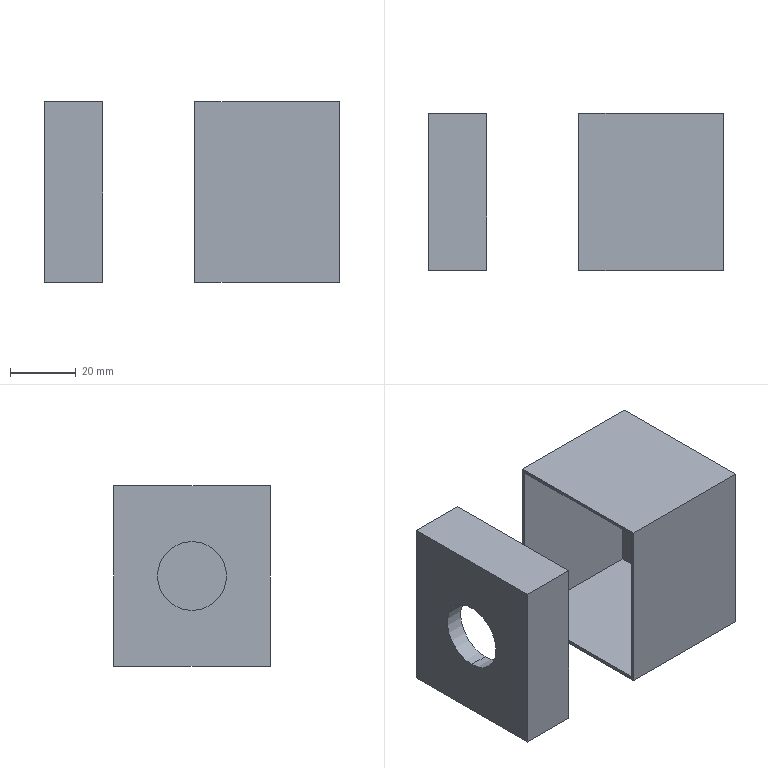Component | SolidWorks | BearingHousing-1 | 2 solids | 24 faces | box 89.77 x 47.79 x 55 mm | volume 29299 mm3 | plane 22 | cylinder 2 | commonest cylinder face diameters 21 x2
STEP:
#1=COLOUR_RGB('',0.7922,0.8196,0.9333);
#2=FILL_AREA_STYLE_COLOUR('',#1);
#3=FILL_AREA_STYLE('',(#2));
#4=SURFACE_STYLE_FILL_AREA(#3);
#5=SURFACE_SIDE_STYLE('',(#4));
#6=SURFACE_STYLE_USAGE(.BOTH.,#5);
#7=PRESENTATION_STYLE_ASSIGNMENT((#6));
#8=CARTESIAN_POINT('',(7.039,3.272,1.043));
#9=VERTEX_POINT('',#8);
#10=CARTESIAN_POINT('',(7.039,1.469,1.043));
#11=VERTEX_POINT('',#10);
#12=CARTESIAN_POINT('',(7.039,3.37,1.043));
#13=DIRECTION('',(0.,-1.,0.));
#14=VECTOR('',#13,39.37);
#15=LINE('',#12,#14);
#16=EDGE_CURVE('',#9,#11,#15,.T.);
#17=ORIENTED_EDGE('',*,*,#16,.T.);
#18=CARTESIAN_POINT('',(7.039,1.469,-1.043));
#19=VERTEX_POINT('',#18);
#20=CARTESIAN_POINT('',(7.039,1.469,0.8331));
#21=DIRECTION('',(-0.,-0.,-1.));
#22=VECTOR('',#21,39.37);
#23=LINE('',#20,#22);
#24=EDGE_CURVE('',#11,#19,#23,.T.);
#25=ORIENTED_EDGE('',*,*,#24,.T.);
#26=CARTESIAN_POINT('',(7.039,3.272,-1.043));
#27=VERTEX_POINT('',#26);
#28=CARTESIAN_POINT('',(7.039,3.37,-1.043));
#29=DIRECTION('',(-0.,1.,-0.));
#30=VECTOR('',#29,39.37);
#31=LINE('',#28,#30);
#32=EDGE_CURVE('',#19,#27,#31,.T.);
#33=ORIENTED_EDGE('',*,*,#32,.T.);
#34=CARTESIAN_POINT('',(7.039,3.272,0.8331));
#35=DIRECTION('',(0.,0.,1.));
#36=VECTOR('',#35,39.37);
#37=LINE('',#34,#36);
#38=EDGE_CURVE('',#27,#9,#37,.T.);
#39=ORIENTED_EDGE('',*,*,#38,.T.);
#40=EDGE_LOOP('',(#17,#25,#33,#39));
#41=FACE_BOUND('',#40,.T.);
#42=CARTESIAN_POINT('',(7.039,1.43,1.083));
#43=VERTEX_POINT('',#42);
#44=CARTESIAN_POINT('',(7.039,1.43,-1.083));
#45=VERTEX_POINT('',#44);
#46=CARTESIAN_POINT('',(7.039,1.43,1.083));
#47=DIRECTION('',(-0.,-0.,-1.));
#48=VECTOR('',#47,39.37);
#49=LINE('',#46,#48);
#50=EDGE_CURVE('',#43,#45,#49,.T.);
#51=ORIENTED_EDGE('',*,*,#50,.F.);
#52=CARTESIAN_POINT('',(7.039,3.312,1.083));
#53=VERTEX_POINT('',#52);
#54=CARTESIAN_POINT('',(7.039,3.312,1.083));
#55=DIRECTION('',(0.,-1.,0.));
#56=VECTOR('',#55,39.37);
#57=LINE('',#54,#56);
#58=EDGE_CURVE('',#53,#43,#57,.T.);
#59=ORIENTED_EDGE('',*,*,#58,.F.);
#60=CARTESIAN_POINT('',(7.039,3.312,-1.083));
#61=VERTEX_POINT('',#60);
#62=CARTESIAN_POINT('',(7.039,3.312,-1.083));
#63=DIRECTION('',(0.,0.,1.));
#64=VECTOR('',#63,39.37);
#65=LINE('',#62,#64);
#66=EDGE_CURVE('',#61,#53,#65,.T.);
#67=ORIENTED_EDGE('',*,*,#66,.F.);
#68=CARTESIAN_POINT('',(7.039,1.43,-1.083));
#69=DIRECTION('',(-0.,1.,-0.));
#70=VECTOR('',#69,39.37);
#71=LINE('',#68,#70);
#72=EDGE_CURVE('',#45,#61,#71,.T.);
#73=ORIENTED_EDGE('',*,*,#72,.F.);
#74=EDGE_LOOP('',(#51,#59,#67,#73));
#75=FACE_OUTER_BOUND('',#74,.T.);
#76=CARTESIAN_POINT('',(7.039,3.37,0.8331));
#77=DIRECTION('',(1.,0.,-0.));
#78=DIRECTION('',(0.,-1.,0.));
#79=AXIS2_PLACEMENT_3D('',#76,#77,#78);
#80=PLANE('',#79);
#81=ADVANCED_FACE('',(#41,#75),#80,.F.);
#82=CARTESIAN_POINT('',(8.771,1.43,-1.083));
#83=VERTEX_POINT('',#82);
#84=CARTESIAN_POINT('',(-2.164,1.43,-1.083));
#85=DIRECTION('',(1.,-0.,0.));
#86=VECTOR('',#85,39.37);
#87=LINE('',#84,#86);
#88=EDGE_CURVE('',#45,#83,#87,.T.);
#89=ORIENTED_EDGE('',*,*,#88,.F.);
#90=ORIENTED_EDGE('',*,*,#72,.T.);
#91=CARTESIAN_POINT('',(8.771,3.312,-1.083));
#92=VERTEX_POINT('',#91);
#93=CARTESIAN_POINT('',(-2.164,3.312,-1.083));
#94=DIRECTION('',(-1.,-0.,-0.));
#95=VECTOR('',#94,39.37);
#96=LINE('',#93,#95);
#97=EDGE_CURVE('',#92,#61,#96,.T.);
#98=ORIENTED_EDGE('',*,*,#97,.F.);
#99=CARTESIAN_POINT('',(8.771,1.43,-1.083));
#100=DIRECTION('',(-0.,1.,-0.));
#101=VECTOR('',#100,39.37);
#102=LINE('',#99,#101);
#103=EDGE_CURVE('',#83,#92,#102,.T.);
#104=ORIENTED_EDGE('',*,*,#103,.F.);
#105=EDGE_LOOP('',(#89,#90,#98,#104));
#106=FACE_OUTER_BOUND('',#105,.T.);
#107=CARTESIAN_POINT('',(-2.164,3.37,-1.083));
#108=DIRECTION('',(-0.,0.,1.));
#109=DIRECTION('',(0.,-1.,0.));
#110=AXIS2_PLACEMENT_3D('',#107,#108,#109);
#111=PLANE('',#110);
#112=ADVANCED_FACE('',(#106),#111,.F.);
#113=ORIENTED_EDGE('',*,*,#58,.T.);
#114=CARTESIAN_POINT('',(8.771,1.43,1.083));
#115=VERTEX_POINT('',#114);
#116=CARTESIAN_POINT('',(-2.164,1.43,1.083));
#117=DIRECTION('',(1.,-0.,0.));
#118=VECTOR('',#117,39.37);
#119=LINE('',#116,#118);
#120=EDGE_CURVE('',#43,#115,#119,.T.);
#121=ORIENTED_EDGE('',*,*,#120,.T.);
#122=CARTESIAN_POINT('',(8.771,3.312,1.083));
#123=VERTEX_POINT('',#122);
#124=CARTESIAN_POINT('',(8.771,3.312,1.083));
#125=DIRECTION('',(0.,-1.,0.));
#126=VECTOR('',#125,39.37);
#127=LINE('',#124,#126);
#128=EDGE_CURVE('',#123,#115,#127,.T.);
#129=ORIENTED_EDGE('',*,*,#128,.F.);
#130=CARTESIAN_POINT('',(-2.164,3.312,1.083));
#131=DIRECTION('',(-1.,-0.,-0.));
#132=VECTOR('',#131,39.37);
#133=LINE('',#130,#132);
#134=EDGE_CURVE('',#123,#53,#133,.T.);
#135=ORIENTED_EDGE('',*,*,#134,.T.);
#136=EDGE_LOOP('',(#113,#121,#129,#135));
#137=FACE_OUTER_BOUND('',#136,.T.);
#138=CARTESIAN_POINT('',(-2.164,3.37,1.083));
#139=DIRECTION('',(-0.,0.,1.));
#140=DIRECTION('',(0.,-1.,0.));
#141=AXIS2_PLACEMENT_3D('',#138,#139,#140);
#142=PLANE('',#141);
#143=ADVANCED_FACE('',(#137),#142,.T.);
#144=ORIENTED_EDGE('',*,*,#120,.F.);
#145=ORIENTED_EDGE('',*,*,#50,.T.);
#146=ORIENTED_EDGE('',*,*,#88,.T.);
#147=CARTESIAN_POINT('',(8.771,1.43,1.083));
#148=DIRECTION('',(-0.,-0.,-1.));
#149=VECTOR('',#148,39.37);
#150=LINE('',#147,#149);
#151=EDGE_CURVE('',#115,#83,#150,.T.);
#152=ORIENTED_EDGE('',*,*,#151,.F.);
#153=EDGE_LOOP('',(#144,#145,#146,#152));
#154=FACE_OUTER_BOUND('',#153,.T.);
#155=CARTESIAN_POINT('',(-2.164,1.43,1.083));
#156=DIRECTION('',(0.,1.,-0.));
#157=DIRECTION('',(0.,0.,1.));
#158=AXIS2_PLACEMENT_3D('',#155,#156,#157);
#159=PLANE('',#158);
#160=ADVANCED_FACE('',(#154),#159,.F.);
#161=ORIENTED_EDGE('',*,*,#97,.T.);
#162=ORIENTED_EDGE('',*,*,#66,.T.);
#163=ORIENTED_EDGE('',*,*,#134,.F.);
#164=CARTESIAN_POINT('',(8.771,3.312,-1.083));
#165=DIRECTION('',(0.,0.,1.));
#166=VECTOR('',#165,39.37);
#167=LINE('',#164,#166);
#168=EDGE_CURVE('',#92,#123,#167,.T.);
#169=ORIENTED_EDGE('',*,*,#168,.F.);
#170=EDGE_LOOP('',(#161,#162,#163,#169));
#171=FACE_OUTER_BOUND('',#170,.T.);
#172=CARTESIAN_POINT('',(-2.164,3.312,1.083));
#173=DIRECTION('',(0.,-1.,0.));
#174=DIRECTION('',(-0.,-0.,-1.));
#175=AXIS2_PLACEMENT_3D('',#172,#173,#174);
#176=PLANE('',#175);
#177=ADVANCED_FACE('',(#171),#176,.F.);
#178=CARTESIAN_POINT('',(8.692,1.469,1.043));
#179=VERTEX_POINT('',#178);
#180=CARTESIAN_POINT('',(8.692,1.469,-1.043));
#181=VERTEX_POINT('',#180);
#182=CARTESIAN_POINT('',(8.692,1.469,1.043));
#183=DIRECTION('',(-0.,-0.,-1.));
#184=VECTOR('',#183,39.37);
#185=LINE('',#182,#184);
#186=EDGE_CURVE('',#179,#181,#185,.T.);
#187=ORIENTED_EDGE('',*,*,#186,.T.);
#188=CARTESIAN_POINT('',(5.464,1.469,-1.043));
#189=DIRECTION('',(1.,0.,0.));
#190=VECTOR('',#189,39.37);
#191=LINE('',#188,#190);
#192=EDGE_CURVE('',#19,#181,#191,.T.);
#193=ORIENTED_EDGE('',*,*,#192,.F.);
#194=ORIENTED_EDGE('',*,*,#24,.F.);
#195=CARTESIAN_POINT('',(5.464,1.469,1.043));
#196=DIRECTION('',(1.,0.,0.));
#197=VECTOR('',#196,39.37);
#198=LINE('',#195,#197);
#199=EDGE_CURVE('',#11,#179,#198,.T.);
#200=ORIENTED_EDGE('',*,*,#199,.T.);
#201=EDGE_LOOP('',(#187,#193,#194,#200));
#202=FACE_OUTER_BOUND('',#201,.T.);
#203=CARTESIAN_POINT('',(5.464,1.469,1.043));
#204=DIRECTION('',(0.,-1.,0.));
#205=DIRECTION('',(-0.,-0.,-1.));
#206=AXIS2_PLACEMENT_3D('',#203,#204,#205);
#207=PLANE('',#206);
#208=ADVANCED_FACE('',(#202),#207,.F.);
#209=CARTESIAN_POINT('',(8.692,3.272,1.043));
#210=VERTEX_POINT('',#209);
#211=CARTESIAN_POINT('',(8.692,3.272,1.043));
#212=DIRECTION('',(0.,-1.,0.));
#213=VECTOR('',#212,39.37);
#214=LINE('',#211,#213);
#215=EDGE_CURVE('',#210,#179,#214,.T.);
#216=ORIENTED_EDGE('',*,*,#215,.T.);
#217=ORIENTED_EDGE('',*,*,#199,.F.);
#218=ORIENTED_EDGE('',*,*,#16,.F.);
#219=CARTESIAN_POINT('',(5.464,3.272,1.043));
#220=DIRECTION('',(1.,0.,0.));
#221=VECTOR('',#220,39.37);
#222=LINE('',#219,#221);
#223=EDGE_CURVE('',#9,#210,#222,.T.);
#224=ORIENTED_EDGE('',*,*,#223,.T.);
#225=EDGE_LOOP('',(#216,#217,#218,#224));
#226=FACE_OUTER_BOUND('',#225,.T.);
#227=CARTESIAN_POINT('',(5.464,3.272,1.043));
#228=DIRECTION('',(-0.,0.,1.));
#229=DIRECTION('',(0.,-1.,0.));
#230=AXIS2_PLACEMENT_3D('',#227,#228,#229);
#231=PLANE('',#230);
#232=ADVANCED_FACE('',(#226),#231,.F.);
#233=CARTESIAN_POINT('',(8.692,3.272,-1.043));
#234=VERTEX_POINT('',#233);
#235=CARTESIAN_POINT('',(8.692,3.272,-1.043));
#236=DIRECTION('',(0.,0.,1.));
#237=VECTOR('',#236,39.37);
#238=LINE('',#235,#237);
#239=EDGE_CURVE('',#234,#210,#238,.T.);
#240=ORIENTED_EDGE('',*,*,#239,.T.);
#241=ORIENTED_EDGE('',*,*,#223,.F.);
#242=ORIENTED_EDGE('',*,*,#38,.F.);
#243=CARTESIAN_POINT('',(5.464,3.272,-1.043));
#244=DIRECTION('',(1.,0.,0.));
#245=VECTOR('',#244,39.37);
#246=LINE('',#243,#245);
#247=EDGE_CURVE('',#27,#234,#246,.T.);
#248=ORIENTED_EDGE('',*,*,#247,.T.);
#249=EDGE_LOOP('',(#240,#241,#242,#248));
#250=FACE_OUTER_BOUND('',#249,.T.);
#251=CARTESIAN_POINT('',(5.464,3.272,-1.043));
#252=DIRECTION('',(-0.,1.,-0.));
#253=DIRECTION('',(0.,0.,1.));
#254=AXIS2_PLACEMENT_3D('',#251,#252,#253);
#255=PLANE('',#254);
#256=ADVANCED_FACE('',(#250),#255,.F.);
#257=CARTESIAN_POINT('',(8.692,1.469,-1.043));
#258=DIRECTION('',(-0.,1.,-0.));
#259=VECTOR('',#258,39.37);
#260=LINE('',#257,#259);
#261=EDGE_CURVE('',#181,#234,#260,.T.);
#262=ORIENTED_EDGE('',*,*,#261,.T.);
#263=ORIENTED_EDGE('',*,*,#247,.F.);
#264=ORIENTED_EDGE('',*,*,#32,.F.);
#265=ORIENTED_EDGE('',*,*,#192,.T.);
#266=EDGE_LOOP('',(#262,#263,#264,#265));
#267=FACE_OUTER_BOUND('',#266,.T.);
#268=CARTESIAN_POINT('',(5.464,1.469,-1.043));
#269=DIRECTION('',(0.,-0.,-1.));
#270=DIRECTION('',(-0.,1.,-0.));
#271=AXIS2_PLACEMENT_3D('',#268,#269,#270);
#272=PLANE('',#271);
#273=ADVANCED_FACE('',(#267),#272,.F.);
#274=ORIENTED_EDGE('',*,*,#151,.T.);
#275=ORIENTED_EDGE('',*,*,#103,.T.);
#276=ORIENTED_EDGE('',*,*,#168,.T.);
#277=ORIENTED_EDGE('',*,*,#128,.T.);
#278=EDGE_LOOP('',(#274,#275,#276,#277));
#279=FACE_OUTER_BOUND('',#278,.T.);
#280=CARTESIAN_POINT('',(8.771,3.37,0.8331));
#281=DIRECTION('',(1.,0.,-0.));
#282=DIRECTION('',(0.,-1.,0.));
#283=AXIS2_PLACEMENT_3D('',#280,#281,#282);
#284=PLANE('',#283);
#285=ADVANCED_FACE('',(#279),#284,.T.);
#286=ORIENTED_EDGE('',*,*,#215,.F.);
#287=ORIENTED_EDGE('',*,*,#239,.F.);
#288=ORIENTED_EDGE('',*,*,#261,.F.);
#289=ORIENTED_EDGE('',*,*,#186,.F.);
#290=EDGE_LOOP('',(#286,#287,#288,#289));
#291=FACE_OUTER_BOUND('',#290,.T.);
#292=CARTESIAN_POINT('',(8.692,3.37,0.8331));
#293=DIRECTION('',(1.,0.,-0.));
#294=DIRECTION('',(0.,-1.,0.));
#295=AXIS2_PLACEMENT_3D('',#292,#293,#294);
#296=PLANE('',#295);
#297=ADVANCED_FACE('',(#291),#296,.F.);
#298=CLOSED_SHELL('',(#81,#112,#143,#160,#177,#208,#232,#256,#273,#285,#297));
#299=MANIFOLD_SOLID_BREP('',#298);
#300=STYLED_ITEM('',(#7),#299);
#301=(LENGTH_UNIT()NAMED_UNIT(*)SI_UNIT($,.METRE.));
#302=LENGTH_MEASURE_WITH_UNIT(LENGTH_MEASURE(0.0254),#301);
#303=DIMENSIONAL_EXPONENTS(1.,0.,0.,0.,0.,0.,0.);
#304=(CONVERSION_BASED_UNIT('',#302)LENGTH_UNIT()NAMED_UNIT(#303));
#305=UNCERTAINTY_MEASURE_WITH_UNIT(LENGTH_MEASURE(0.00001),#304,'','');
#306=(NAMED_UNIT(*)PLANE_ANGLE_UNIT()SI_UNIT($,.RADIAN.));
#307=(NAMED_UNIT(*)SI_UNIT($,.STERADIAN.)SOLID_ANGLE_UNIT());
#308=(GEOMETRIC_REPRESENTATION_CONTEXT(3)GLOBAL_UNCERTAINTY_ASSIGNED_CONTEXT((#305))GLOBAL_UNIT_ASSIGNED_CONTEXT((#304,#306,#307))REPRESENTATION_CONTEXT('',''));
#309=MECHANICAL_DESIGN_GEOMETRIC_PRESENTATION_REPRESENTATION('',(#300),#308);
#310=COLOUR_RGB('',0.7922,0.8196,0.9333);
#311=FILL_AREA_STYLE_COLOUR('',#310);
#312=FILL_AREA_STYLE('',(#311));
#313=SURFACE_STYLE_FILL_AREA(#312);
#314=SURFACE_SIDE_STYLE('',(#313));
#315=SURFACE_STYLE_USAGE(.BOTH.,#314);
#316=PRESENTATION_STYLE_ASSIGNMENT((#315));
#317=CARTESIAN_POINT('',(5.464,2.371,-0.4134));
#318=VERTEX_POINT('',#317);
#319=CARTESIAN_POINT('',(5.464,2.371,0.4134));
#320=VERTEX_POINT('',#319);
#321=CARTESIAN_POINT('',(5.464,2.371,-0.));
#322=DIRECTION('',(-1.,-0.,0.));
#323=DIRECTION('',(0.,-1.,0.));
#324=AXIS2_PLACEMENT_3D('',#321,#322,#323);
#325=CIRCLE('',#324,0.4134);
#326=EDGE_CURVE('',#318,#320,#325,.T.);
#327=ORIENTED_EDGE('',*,*,#326,.F.);
#328=CARTESIAN_POINT('',(5.237,2.371,-0.4134));
#329=VERTEX_POINT('',#328);
#330=CARTESIAN_POINT('',(7.639,2.371,-0.4134));
#331=DIRECTION('',(-1.,-0.,-0.));
#332=VECTOR('',#331,39.37);
#333=LINE('',#330,#332);
#334=EDGE_CURVE('',#318,#329,#333,.T.);
#335=ORIENTED_EDGE('',*,*,#334,.T.);
#336=CARTESIAN_POINT('',(5.237,2.371,0.4134));
#337=VERTEX_POINT('',#336);
#338=CARTESIAN_POINT('',(5.237,2.371,-0.));
#339=DIRECTION('',(-1.,-0.,-0.));
#340=DIRECTION('',(0.,0.,1.));
#341=AXIS2_PLACEMENT_3D('',#338,#339,#340);
#342=CIRCLE('',#341,0.4134);
#343=EDGE_CURVE('',#329,#337,#342,.T.);
#344=ORIENTED_EDGE('',*,*,#343,.T.);
#345=CARTESIAN_POINT('',(7.639,2.371,0.4134));
#346=DIRECTION('',(-1.,-0.,-0.));
#347=VECTOR('',#346,39.37);
#348=LINE('',#345,#347);
#349=EDGE_CURVE('',#320,#337,#348,.T.);
#350=ORIENTED_EDGE('',*,*,#349,.F.);
#351=EDGE_LOOP('',(#327,#335,#344,#350));
#352=FACE_OUTER_BOUND('',#351,.T.);
#353=CARTESIAN_POINT('',(7.639,2.371,0.));
#354=DIRECTION('',(-1.,-0.,-0.));
#355=DIRECTION('',(0.,0.,1.));
#356=AXIS2_PLACEMENT_3D('',#353,#354,#355);
#357=CYLINDRICAL_SURFACE('',#356,0.4134);
#358=ADVANCED_FACE('',(#352),#357,.F.);
#359=CARTESIAN_POINT('',(5.237,1.43,1.083));
#360=VERTEX_POINT('',#359);
#361=CARTESIAN_POINT('',(5.936,1.43,1.083));
#362=VERTEX_POINT('',#361);
#363=CARTESIAN_POINT('',(-2.164,1.43,1.083));
#364=DIRECTION('',(1.,-0.,0.));
#365=VECTOR('',#364,39.37);
#366=LINE('',#363,#365);
#367=EDGE_CURVE('',#360,#362,#366,.T.);
#368=ORIENTED_EDGE('',*,*,#367,.T.);
#369=CARTESIAN_POINT('',(5.936,3.312,1.083));
#370=VERTEX_POINT('',#369);
#371=CARTESIAN_POINT('',(5.936,3.312,1.083));
#372=DIRECTION('',(0.,-1.,0.));
#373=VECTOR('',#372,39.37);
#374=LINE('',#371,#373);
#375=EDGE_CURVE('',#370,#362,#374,.T.);
#376=ORIENTED_EDGE('',*,*,#375,.F.);
#377=CARTESIAN_POINT('',(5.237,3.312,1.083));
#378=VERTEX_POINT('',#377);
#379=CARTESIAN_POINT('',(-2.164,3.312,1.083));
#380=DIRECTION('',(-1.,-0.,-0.));
#381=VECTOR('',#380,39.37);
#382=LINE('',#379,#381);
#383=EDGE_CURVE('',#370,#378,#382,.T.);
#384=ORIENTED_EDGE('',*,*,#383,.T.);
#385=CARTESIAN_POINT('',(5.237,3.37,1.083));
#386=DIRECTION('',(0.,-1.,0.));
#387=VECTOR('',#386,39.37);
#388=LINE('',#385,#387);
#389=EDGE_CURVE('',#378,#360,#388,.T.);
#390=ORIENTED_EDGE('',*,*,#389,.T.);
#391=EDGE_LOOP('',(#368,#376,#384,#390));
#392=FACE_OUTER_BOUND('',#391,.T.);
#393=CARTESIAN_POINT('',(-2.164,3.37,1.083));
#394=DIRECTION('',(-0.,0.,1.));
#395=DIRECTION('',(0.,-1.,0.));
#396=AXIS2_PLACEMENT_3D('',#393,#394,#395);
#397=PLANE('',#396);
#398=ADVANCED_FACE('',(#392),#397,.T.);
#399=CARTESIAN_POINT('',(5.936,3.312,-1.083));
#400=VERTEX_POINT('',#399);
#401=CARTESIAN_POINT('',(5.936,3.312,-1.083));
#402=DIRECTION('',(0.,0.,1.));
#403=VECTOR('',#402,39.37);
#404=LINE('',#401,#403);
#405=EDGE_CURVE('',#400,#370,#404,.T.);
#406=ORIENTED_EDGE('',*,*,#405,.F.);
#407=CARTESIAN_POINT('',(5.237,3.312,-1.083));
#408=VERTEX_POINT('',#407);
#409=CARTESIAN_POINT('',(-2.164,3.312,-1.083));
#410=DIRECTION('',(-1.,-0.,-0.));
#411=VECTOR('',#410,39.37);
#412=LINE('',#409,#411);
#413=EDGE_CURVE('',#400,#408,#412,.T.);
#414=ORIENTED_EDGE('',*,*,#413,.T.);
#415=CARTESIAN_POINT('',(5.237,3.312,1.083));
#416=DIRECTION('',(0.,-0.,-1.));
#417=VECTOR('',#416,39.37);
#418=LINE('',#415,#417);
#419=EDGE_CURVE('',#378,#408,#418,.T.);
#420=ORIENTED_EDGE('',*,*,#419,.F.);
#421=ORIENTED_EDGE('',*,*,#383,.F.);
#422=EDGE_LOOP('',(#406,#414,#420,#421));
#423=FACE_OUTER_BOUND('',#422,.T.);
#424=CARTESIAN_POINT('',(-2.164,3.312,1.083));
#425=DIRECTION('',(0.,-1.,0.));
#426=DIRECTION('',(-0.,-0.,-1.));
#427=AXIS2_PLACEMENT_3D('',#424,#425,#426);
#428=PLANE('',#427);
#429=ADVANCED_FACE('',(#423),#428,.F.);
#430=CARTESIAN_POINT('',(5.936,1.43,-1.083));
#431=VERTEX_POINT('',#430);
#432=CARTESIAN_POINT('',(5.936,1.43,-1.083));
#433=DIRECTION('',(-0.,1.,-0.));
#434=VECTOR('',#433,39.37);
#435=LINE('',#432,#434);
#436=EDGE_CURVE('',#431,#400,#435,.T.);
#437=ORIENTED_EDGE('',*,*,#436,.F.);
#438=CARTESIAN_POINT('',(5.237,1.43,-1.083));
#439=VERTEX_POINT('',#438);
#440=CARTESIAN_POINT('',(-2.164,1.43,-1.083));
#441=DIRECTION('',(1.,-0.,0.));
#442=VECTOR('',#441,39.37);
#443=LINE('',#440,#442);
#444=EDGE_CURVE('',#439,#431,#443,.T.);
#445=ORIENTED_EDGE('',*,*,#444,.F.);
#446=CARTESIAN_POINT('',(5.237,3.37,-1.083));
#447=DIRECTION('',(0.,-1.,0.));
#448=VECTOR('',#447,39.37);
#449=LINE('',#446,#448);
#450=EDGE_CURVE('',#408,#439,#449,.T.);
#451=ORIENTED_EDGE('',*,*,#450,.F.);
#452=ORIENTED_EDGE('',*,*,#413,.F.);
#453=EDGE_LOOP('',(#437,#445,#451,#452));
#454=FACE_OUTER_BOUND('',#453,.T.);
#455=CARTESIAN_POINT('',(-2.164,3.37,-1.083));
#456=DIRECTION('',(-0.,0.,1.));
#457=DIRECTION('',(0.,-1.,0.));
#458=AXIS2_PLACEMENT_3D('',#455,#456,#457);
#459=PLANE('',#458);
#460=ADVANCED_FACE('',(#454),#459,.F.);
#461=CARTESIAN_POINT('',(5.237,2.371,-0.));
#462=DIRECTION('',(-1.,-0.,-0.));
#463=DIRECTION('',(0.,0.,1.));
#464=AXIS2_PLACEMENT_3D('',#461,#462,#463);
#465=CIRCLE('',#464,0.4134);
#466=EDGE_CURVE('',#337,#329,#465,.T.);
#467=ORIENTED_EDGE('',*,*,#466,.F.);
#468=ORIENTED_EDGE('',*,*,#343,.F.);
#469=EDGE_LOOP('',(#467,#468));
#470=FACE_BOUND('',#469,.T.);
#471=ORIENTED_EDGE('',*,*,#450,.T.);
#472=CARTESIAN_POINT('',(5.237,1.43,1.083));
#473=DIRECTION('',(0.,-0.,-1.));
#474=VECTOR('',#473,39.37);
#475=LINE('',#472,#474);
#476=EDGE_CURVE('',#360,#439,#475,.T.);
#477=ORIENTED_EDGE('',*,*,#476,.F.);
#478=ORIENTED_EDGE('',*,*,#389,.F.);
#479=ORIENTED_EDGE('',*,*,#419,.T.);
#480=EDGE_LOOP('',(#471,#477,#478,#479));
#481=FACE_OUTER_BOUND('',#480,.T.);
#482=CARTESIAN_POINT('',(5.237,3.37,1.083));
#483=DIRECTION('',(1.,0.,0.));
#484=DIRECTION('',(0.,-0.,-1.));
#485=AXIS2_PLACEMENT_3D('',#482,#483,#484);
#486=PLANE('',#485);
#487=ADVANCED_FACE('',(#470,#481),#486,.F.);
#488=ORIENTED_EDGE('',*,*,#334,.F.);
#489=CARTESIAN_POINT('',(5.464,2.371,-0.));
#490=DIRECTION('',(-1.,-0.,0.));
#491=DIRECTION('',(0.,-1.,0.));
#492=AXIS2_PLACEMENT_3D('',#489,#490,#491);
#493=CIRCLE('',#492,0.4134);
#494=EDGE_CURVE('',#320,#318,#493,.T.);
#495=ORIENTED_EDGE('',*,*,#494,.F.);
#496=ORIENTED_EDGE('',*,*,#349,.T.);
#497=ORIENTED_EDGE('',*,*,#466,.T.);
#498=EDGE_LOOP('',(#488,#495,#496,#497));
#499=FACE_OUTER_BOUND('',#498,.T.);
#500=CARTESIAN_POINT('',(7.639,2.371,0.));
#501=DIRECTION('',(-1.,-0.,-0.));
#502=DIRECTION('',(0.,0.,1.));
#503=AXIS2_PLACEMENT_3D('',#500,#501,#502);
#504=CYLINDRICAL_SURFACE('',#503,0.4134);
#505=ADVANCED_FACE('',(#499),#504,.F.);
#506=CARTESIAN_POINT('',(5.936,1.43,1.083));
#507=DIRECTION('',(-0.,-0.,-1.));
#508=VECTOR('',#507,39.37);
#509=LINE('',#506,#508);
#510=EDGE_CURVE('',#362,#431,#509,.T.);
#511=ORIENTED_EDGE('',*,*,#510,.F.);
#512=ORIENTED_EDGE('',*,*,#367,.F.);
#513=ORIENTED_EDGE('',*,*,#476,.T.);
#514=ORIENTED_EDGE('',*,*,#444,.T.);
#515=EDGE_LOOP('',(#511,#512,#513,#514));
#516=FACE_OUTER_BOUND('',#515,.T.);
#517=CARTESIAN_POINT('',(-2.164,1.43,1.083));
#518=DIRECTION('',(0.,1.,-0.));
#519=DIRECTION('',(0.,0.,1.));
#520=AXIS2_PLACEMENT_3D('',#517,#518,#519);
#521=PLANE('',#520);
#522=ADVANCED_FACE('',(#516),#521,.F.);
#523=CARTESIAN_POINT('',(5.936,1.469,1.043));
#524=VERTEX_POINT('',#523);
#525=CARTESIAN_POINT('',(5.936,1.469,-1.043));
#526=VERTEX_POINT('',#525);
#527=CARTESIAN_POINT('',(5.936,1.469,0.8331));
#528=DIRECTION('',(-0.,-0.,-1.));
#529=VECTOR('',#528,39.37);
#530=LINE('',#527,#529);
#531=EDGE_CURVE('',#524,#526,#530,.T.);
#532=ORIENTED_EDGE('',*,*,#531,.F.);
#533=CARTESIAN_POINT('',(5.936,3.272,1.043));
#534=VERTEX_POINT('',#533);
#535=CARTESIAN_POINT('',(5.936,3.37,1.043));
#536=DIRECTION('',(0.,-1.,0.));
#537=VECTOR('',#536,39.37);
#538=LINE('',#535,#537);
#539=EDGE_CURVE('',#534,#524,#538,.T.);
#540=ORIENTED_EDGE('',*,*,#539,.F.);
#541=CARTESIAN_POINT('',(5.936,3.272,-1.043));
#542=VERTEX_POINT('',#541);
#543=CARTESIAN_POINT('',(5.936,3.272,0.8331));
#544=DIRECTION('',(0.,0.,1.));
#545=VECTOR('',#544,39.37);
#546=LINE('',#543,#545);
#547=EDGE_CURVE('',#542,#534,#546,.T.);
#548=ORIENTED_EDGE('',*,*,#547,.F.);
#549=CARTESIAN_POINT('',(5.936,3.37,-1.043));
#550=DIRECTION('',(-0.,1.,-0.));
#551=VECTOR('',#550,39.37);
#552=LINE('',#549,#551);
#553=EDGE_CURVE('',#526,#542,#552,.T.);
#554=ORIENTED_EDGE('',*,*,#553,.F.);
#555=EDGE_LOOP('',(#532,#540,#548,#554));
#556=FACE_BOUND('',#555,.T.);
#557=ORIENTED_EDGE('',*,*,#510,.T.);
#558=ORIENTED_EDGE('',*,*,#436,.T.);
#559=ORIENTED_EDGE('',*,*,#405,.T.);
#560=ORIENTED_EDGE('',*,*,#375,.T.);
#561=EDGE_LOOP('',(#557,#558,#559,#560));
#562=FACE_OUTER_BOUND('',#561,.T.);
#563=CARTESIAN_POINT('',(5.936,3.37,0.8331));
#564=DIRECTION('',(1.,0.,-0.));
#565=DIRECTION('',(0.,-1.,0.));
#566=AXIS2_PLACEMENT_3D('',#563,#564,#565);
#567=PLANE('',#566);
#568=ADVANCED_FACE('',(#556,#562),#567,.T.);
#569=CARTESIAN_POINT('',(5.464,1.469,1.043));
#570=VERTEX_POINT('',#569);
#571=CARTESIAN_POINT('',(5.464,1.469,-1.043));
#572=VERTEX_POINT('',#571);
#573=CARTESIAN_POINT('',(5.464,1.469,1.043));
#574=DIRECTION('',(-0.,-0.,-1.));
#575=VECTOR('',#574,39.37);
#576=LINE('',#573,#575);
#577=EDGE_CURVE('',#570,#572,#576,.T.);
#578=ORIENTED_EDGE('',*,*,#577,.T.);
#579=CARTESIAN_POINT('',(5.464,3.272,-1.043));
#580=VERTEX_POINT('',#579);
#581=CARTESIAN_POINT('',(5.464,1.469,-1.043));
#582=DIRECTION('',(-0.,1.,-0.));
#583=VECTOR('',#582,39.37);
#584=LINE('',#581,#583);
#585=EDGE_CURVE('',#572,#580,#584,.T.);
#586=ORIENTED_EDGE('',*,*,#585,.T.);
#587=CARTESIAN_POINT('',(5.464,3.272,1.043));
#588=VERTEX_POINT('',#587);
#589=CARTESIAN_POINT('',(5.464,3.272,-1.043));
#590=DIRECTION('',(0.,0.,1.));
#591=VECTOR('',#590,39.37);
#592=LINE('',#589,#591);
#593=EDGE_CURVE('',#580,#588,#592,.T.);
#594=ORIENTED_EDGE('',*,*,#593,.T.);
#595=CARTESIAN_POINT('',(5.464,3.272,1.043));
#596=DIRECTION('',(0.,-1.,0.));
#597=VECTOR('',#596,39.37);
#598=LINE('',#595,#597);
#599=EDGE_CURVE('',#588,#570,#598,.T.);
#600=ORIENTED_EDGE('',*,*,#599,.T.);
#601=EDGE_LOOP('',(#578,#586,#594,#600));
#602=FACE_OUTER_BOUND('',#601,.T.);
#603=ORIENTED_EDGE('',*,*,#494,.T.);
#604=ORIENTED_EDGE('',*,*,#326,.T.);
#605=EDGE_LOOP('',(#603,#604));
#606=FACE_BOUND('',#605,.T.);
#607=CARTESIAN_POINT('',(5.464,3.37,0.8331));
#608=DIRECTION('',(1.,0.,-0.));
#609=DIRECTION('',(0.,-1.,0.));
#610=AXIS2_PLACEMENT_3D('',#607,#608,#609);
#611=PLANE('',#610);
#612=ADVANCED_FACE('',(#602,#606),#611,.T.);
#613=ORIENTED_EDGE('',*,*,#553,.T.);
#614=CARTESIAN_POINT('',(5.464,3.272,-1.043));
#615=DIRECTION('',(1.,0.,0.));
#616=VECTOR('',#615,39.37);
#617=LINE('',#614,#616);
#618=EDGE_CURVE('',#580,#542,#617,.T.);
#619=ORIENTED_EDGE('',*,*,#618,.F.);
#620=ORIENTED_EDGE('',*,*,#585,.F.);
#621=CARTESIAN_POINT('',(5.464,1.469,-1.043));
#622=DIRECTION('',(1.,0.,0.));
#623=VECTOR('',#622,39.37);
#624=LINE('',#621,#623);
#625=EDGE_CURVE('',#572,#526,#624,.T.);
#626=ORIENTED_EDGE('',*,*,#625,.T.);
#627=EDGE_LOOP('',(#613,#619,#620,#626));
#628=FACE_OUTER_BOUND('',#627,.T.);
#629=CARTESIAN_POINT('',(5.464,1.469,-1.043));
#630=DIRECTION('',(0.,-0.,-1.));
#631=DIRECTION('',(-0.,1.,-0.));
#632=AXIS2_PLACEMENT_3D('',#629,#630,#631);
#633=PLANE('',#632);
#634=ADVANCED_FACE('',(#628),#633,.F.);
#635=ORIENTED_EDGE('',*,*,#547,.T.);
#636=CARTESIAN_POINT('',(5.464,3.272,1.043));
#637=DIRECTION('',(1.,0.,0.));
#638=VECTOR('',#637,39.37);
#639=LINE('',#636,#638);
#640=EDGE_CURVE('',#588,#534,#639,.T.);
#641=ORIENTED_EDGE('',*,*,#640,.F.);
#642=ORIENTED_EDGE('',*,*,#593,.F.);
#643=ORIENTED_EDGE('',*,*,#618,.T.);
#644=EDGE_LOOP('',(#635,#641,#642,#643));
#645=FACE_OUTER_BOUND('',#644,.T.);
#646=CARTESIAN_POINT('',(5.464,3.272,-1.043));
#647=DIRECTION('',(-0.,1.,-0.));
#648=DIRECTION('',(0.,0.,1.));
#649=AXIS2_PLACEMENT_3D('',#646,#647,#648);
#650=PLANE('',#649);
#651=ADVANCED_FACE('',(#645),#650,.F.);
#652=ORIENTED_EDGE('',*,*,#539,.T.);
#653=CARTESIAN_POINT('',(5.464,1.469,1.043));
#654=DIRECTION('',(1.,0.,0.));
#655=VECTOR('',#654,39.37);
#656=LINE('',#653,#655);
#657=EDGE_CURVE('',#570,#524,#656,.T.);
#658=ORIENTED_EDGE('',*,*,#657,.F.);
#659=ORIENTED_EDGE('',*,*,#599,.F.);
#660=ORIENTED_EDGE('',*,*,#640,.T.);
#661=EDGE_LOOP('',(#652,#658,#659,#660));
#662=FACE_OUTER_BOUND('',#661,.T.);
#663=CARTESIAN_POINT('',(5.464,3.272,1.043));
#664=DIRECTION('',(-0.,0.,1.));
#665=DIRECTION('',(0.,-1.,0.));
#666=AXIS2_PLACEMENT_3D('',#663,#664,#665);
#667=PLANE('',#666);
#668=ADVANCED_FACE('',(#662),#667,.F.);
#669=ORIENTED_EDGE('',*,*,#531,.T.);
#670=ORIENTED_EDGE('',*,*,#625,.F.);
#671=ORIENTED_EDGE('',*,*,#577,.F.);
#672=ORIENTED_EDGE('',*,*,#657,.T.);
#673=EDGE_LOOP('',(#669,#670,#671,#672));
#674=FACE_OUTER_BOUND('',#673,.T.);
#675=CARTESIAN_POINT('',(5.464,1.469,1.043));
#676=DIRECTION('',(0.,-1.,0.));
#677=DIRECTION('',(-0.,-0.,-1.));
#678=AXIS2_PLACEMENT_3D('',#675,#676,#677);
#679=PLANE('',#678);
#680=ADVANCED_FACE('',(#674),#679,.F.);
#681=CLOSED_SHELL('',(#358,#398,#429,#460,#487,#505,#522,#568,#612,#634,#651,#668,#680));
#682=MANIFOLD_SOLID_BREP('',#681);
#683=STYLED_ITEM('',(#316),#682);
#684=PRESENTATION_LAYER_ASSIGNMENT('','',(#683));
#685=(LENGTH_UNIT()NAMED_UNIT(*)SI_UNIT($,.METRE.));
#686=LENGTH_MEASURE_WITH_UNIT(LENGTH_MEASURE(0.0254),#685);
#687=DIMENSIONAL_EXPONENTS(1.,0.,0.,0.,0.,0.,0.);
#688=(CONVERSION_BASED_UNIT('',#686)LENGTH_UNIT()NAMED_UNIT(#687));
#689=UNCERTAINTY_MEASURE_WITH_UNIT(LENGTH_MEASURE(0.00001),#688,'','');
#690=(NAMED_UNIT(*)PLANE_ANGLE_UNIT()SI_UNIT($,.RADIAN.));
#691=(NAMED_UNIT(*)SI_UNIT($,.STERADIAN.)SOLID_ANGLE_UNIT());
#692=(GEOMETRIC_REPRESENTATION_CONTEXT(3)GLOBAL_UNCERTAINTY_ASSIGNED_CONTEXT((#689))GLOBAL_UNIT_ASSIGNED_CONTEXT((#688,#690,#691))REPRESENTATION_CONTEXT('',''));
#693=MECHANICAL_DESIGN_GEOMETRIC_PRESENTATION_REPRESENTATION('',(#683),#692);
#694=CARTESIAN_POINT('',(0.,0.,0.));
#695=DIRECTION('',(0.,0.,1.));
#696=DIRECTION('',(1.,0.,0.));
#697=AXIS2_PLACEMENT_3D('',#694,#695,#696);
#698=(LENGTH_UNIT()NAMED_UNIT(*)SI_UNIT($,.METRE.));
#699=LENGTH_MEASURE_WITH_UNIT(LENGTH_MEASURE(0.0254),#698);
#700=DIMENSIONAL_EXPONENTS(1.,0.,0.,0.,0.,0.,0.);
#701=(CONVERSION_BASED_UNIT('',#699)LENGTH_UNIT()NAMED_UNIT(#700));
#702=UNCERTAINTY_MEASURE_WITH_UNIT(LENGTH_MEASURE(0.00001),#701,'','');
#703=(NAMED_UNIT(*)PLANE_ANGLE_UNIT()SI_UNIT($,.RADIAN.));
#704=(NAMED_UNIT(*)SI_UNIT($,.STERADIAN.)SOLID_ANGLE_UNIT());
#705=(GEOMETRIC_REPRESENTATION_CONTEXT(3)GLOBAL_UNCERTAINTY_ASSIGNED_CONTEXT((#702))GLOBAL_UNIT_ASSIGNED_CONTEXT((#701,#703,#704))REPRESENTATION_CONTEXT('',''));
#706=ADVANCED_BREP_SHAPE_REPRESENTATION('',(#299,#682,#697),#705);
#707=PRESENTATION_LAYER_ASSIGNMENT('','',(#300));